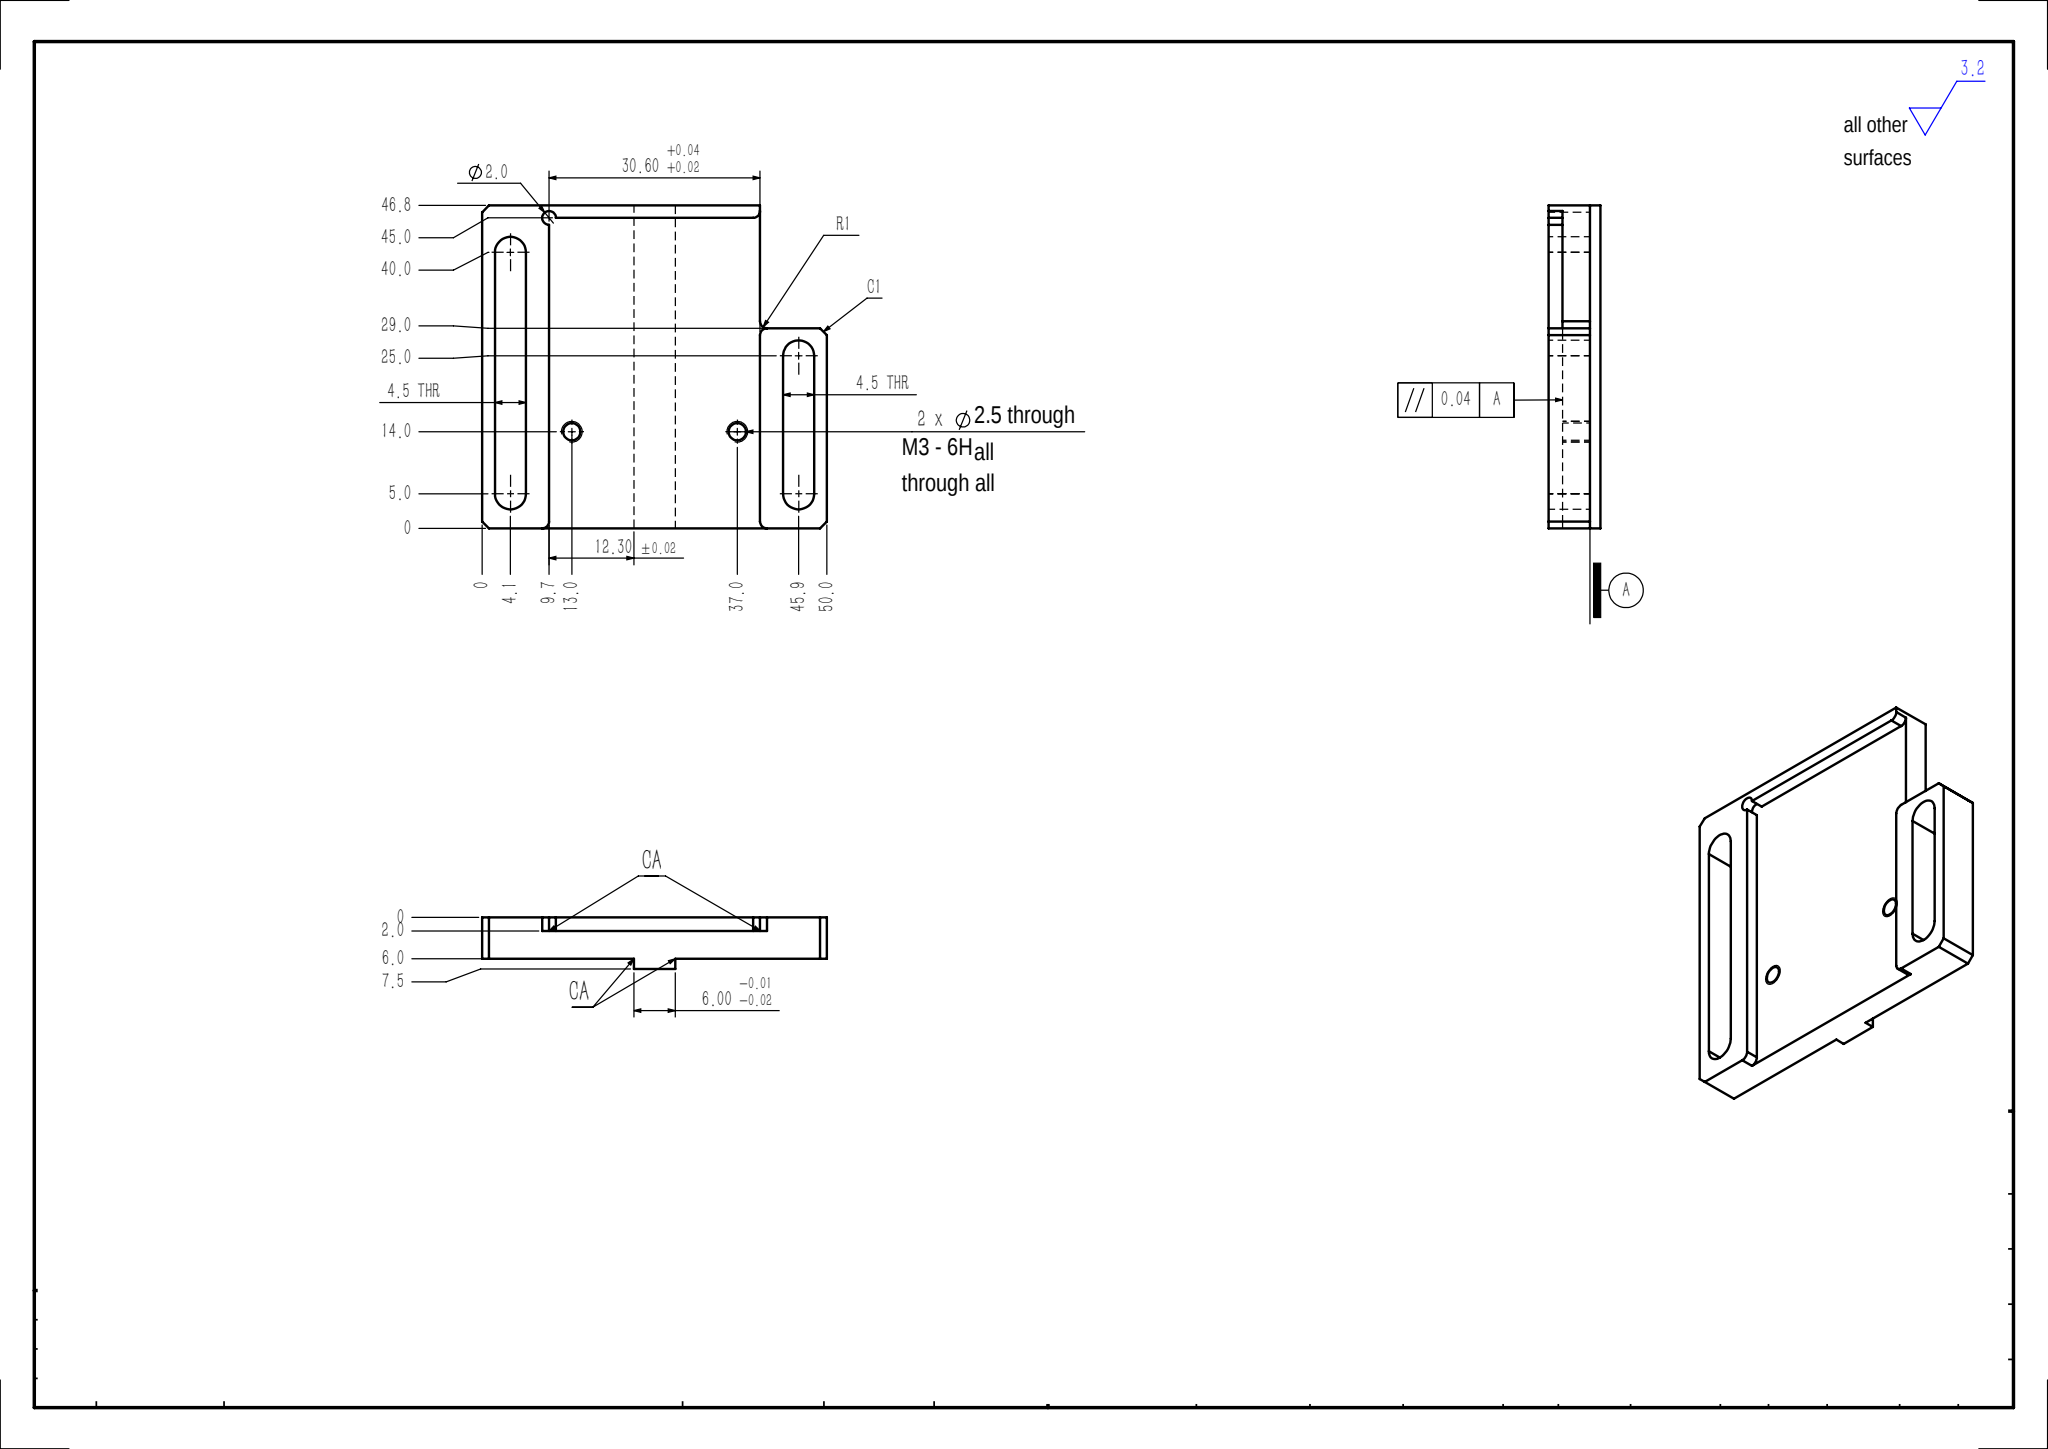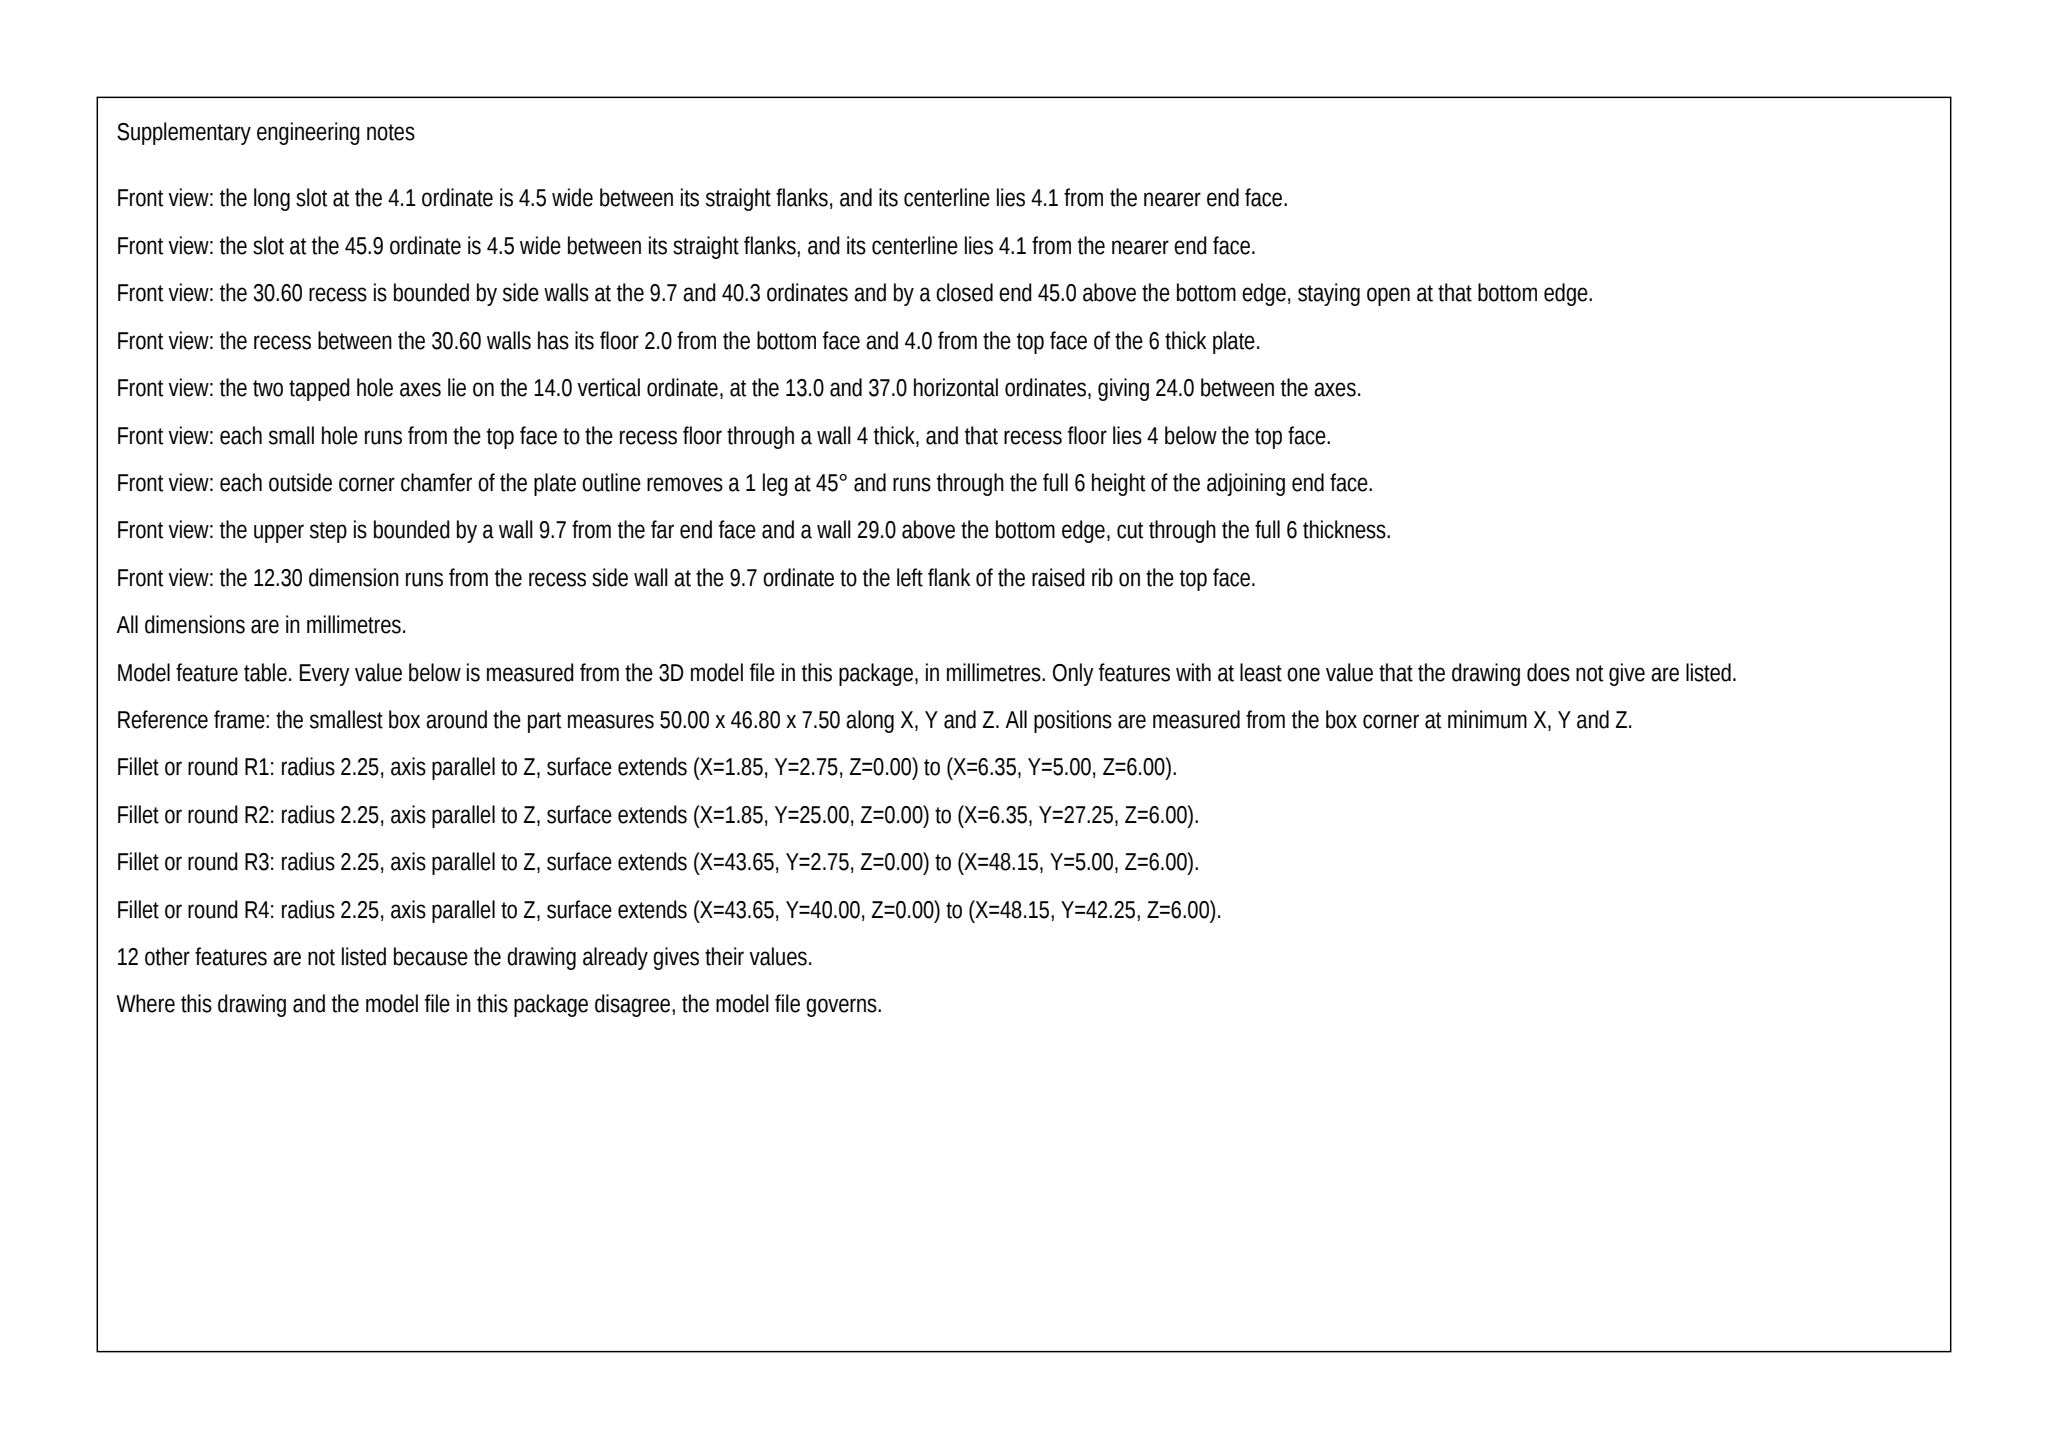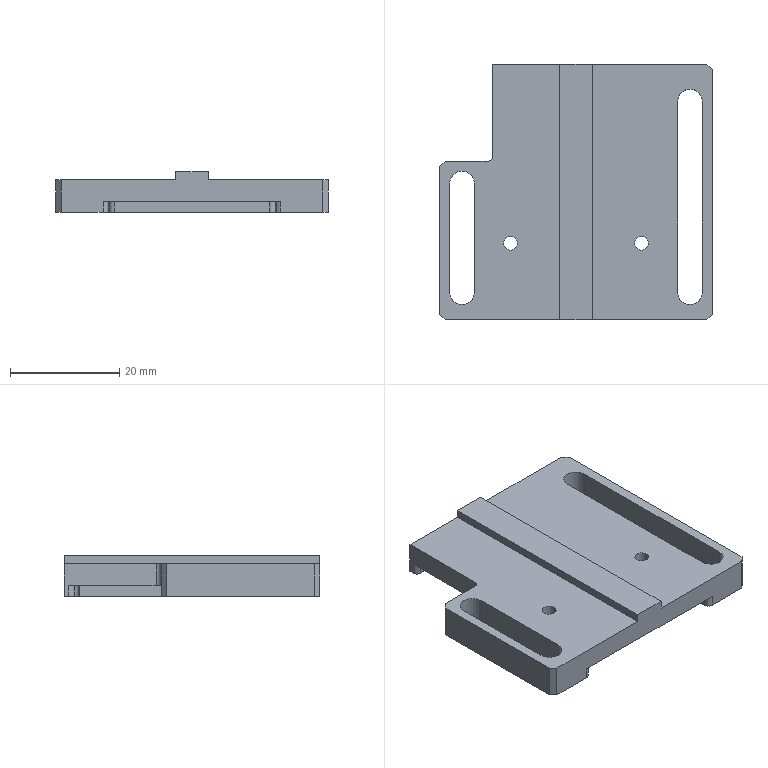Part | SolidWorks | mm | 1 solid | 40 faces | box 50 x 46.8 x 7.5 mm | volume 8939 mm3 | plane 25 | cylinder 15 | commonest cylinder face diameters 2 x7 2.5 x4 4.5 x4
Drawing notes:
6X Ø2.0 CORNER RELIEF CUTS (CA) | from the solid: Six Ø2.0 z-axis cylinders at (8.7,1.0),(8.7,28.0),(8.7,30.0),(10.7,46.0),(40.3,45.0),(41.3,1.0)
Ø2.0 RELIEF CL: Y=1.0, 28.0, 30.0, 45.0, 46.0 FROM Y0 | from the solid: Ø2.0 cylinder pos_other_axes y values 1.0, 28.0, 30.0, 45.0, 46.0 from bbox min y (drawing 0 datum)
Ø2.0 RELIEF X CL: 8.7, 10.7, 40.3, 41.3 FROM X0 | from the solid: Ø2.0 cylinder x positions 8.7, 10.7, 40.3, 41.3 from bbox min x (drawing 0 datum)
Ø2.0 RELIEF DP 2.0 TYP; DP 4.0 AT X8.7 / Y30.0 | from the solid: Ø2.0 cylinder lengths: 2.0 for five, 4.0 for the one at (8.7,30.0)
CA = Ø2.0 CORNER RELIEF, DP 2.0 UNO, SEE FRONT VIEW | from the solid: CA labels in section coincide with Ø2.0 z-axis relief cylinders, length 2.0
RELIEF AXIAL LEN 2.0 AT X9.7 & X40.3 STEP EDGES | from the solid: Ø2.0 cylinders tangent to planes x=9.7 and x=40.3, cylinder length 2.0
build123d program:
from build123d import *

# Parameters (mm, degrees)
SKETCH1_W           = 50
SKETCH1_H           = 47
BOSS_EXTRUDE1_DEPTH = 3
SKETCH2_W           = 30.6
SKETCH2_H           = 45
CUT_EXTRUDE1_DEPTH  = 2
SKETCH3_R           = 1
CUT_EXTRUDE2_DEPTH  = 35.543
SKETCH4_W           = 9.7
SKETCH4_H           = 18
CUT_EXTRUDE3_DEPTH  = 35.832
CUT_EXTRUDE4_DEPTH  = 35.832
SKETCH6_W           = 40.3
SKETCH6_H           = 6
CUT_EXTRUDE5_DEPTH  = 0.2
M3_TAPPED_HOLE1_D   = 2.5
SKETCH9_W           = 6
SKETCH9_H           = 46.8
BOSS_EXTRUDE2_DEPTH = 1.5
FILLET1_R           = 1
FILLET2_R           = 1
CHAMFER1_SIZE       = 1


with BuildPart() as part:
    # Sketch1 → Boss-Extrude1 (new, symmetric)
    with BuildSketch(Plane.XY):
        Rectangle(SKETCH1_W, SKETCH1_H)
    extrude(amount=BOSS_EXTRUDE1_DEPTH, both=True)

    # Sketch2 → Cut-Extrude1 (cut)
    with BuildSketch(Plane(origin=(0, 0, -3), x_dir=(-1, 0, 0), z_dir=(0, 0, -1))):
        with Locations((0, -1)):
            Rectangle(SKETCH2_W, SKETCH2_H)
    extrude(amount=-CUT_EXTRUDE1_DEPTH, mode=Mode.SUBTRACT)

    # Sketch3 → Cut-Extrude2 (cut, through all)
    with BuildSketch(Plane(origin=(0, 0, -1), x_dir=(-1, 0, 0), z_dir=(0, 0, -1))):
        with Locations((-15.3, 21.5)):
            Circle(SKETCH3_R)
    extrude(amount=CUT_EXTRUDE2_DEPTH, mode=Mode.SUBTRACT)

    # Sketch4 → Cut-Extrude3 (cut, through all)
    with BuildSketch(Plane(origin=(0, 0, -3), x_dir=(-1, 0, 0), z_dir=(0, 0, -1))):
        with Locations((20.15, 14.5)):
            Rectangle(SKETCH4_W, SKETCH4_H)
    extrude(amount=-CUT_EXTRUDE3_DEPTH, mode=Mode.SUBTRACT)

    # Sketch5 → Cut-Extrude4 (cut, through all)
    with BuildSketch(Plane(origin=(0, 0, -3), x_dir=(-1, 0, 0), z_dir=(0, 0, -1))):
        with BuildLine():
            Line((18.65, -18.5), (18.65, 1.5))
            ThreePointArc((18.65, 1.5), (20.9, 3.75), (23.15, 1.5))
            Line((23.15, 1.5), (23.15, -18.5))
            ThreePointArc((23.15, -18.5), (20.9, -20.75), (18.65, -18.5))
        make_face()
        with BuildLine():
            Line((-23.15, -18.5), (-23.15, 16.5))
            ThreePointArc((-23.15, 16.5), (-20.9, 18.75), (-18.65, 16.5))
            Line((-18.65, 16.5), (-18.65, -18.5))
            ThreePointArc((-18.65, -18.5), (-20.9, -20.75), (-23.15, -18.5))
        make_face()
    extrude(amount=-CUT_EXTRUDE4_DEPTH, mode=Mode.SUBTRACT)

    # Sketch6 → Cut-Extrude5 (cut)
    with BuildSketch(Plane(origin=(0, 23.5, 0), x_dir=(1, 0, 0), z_dir=(0, 1, 0))):
        with Locations((4.85, 0)):
            Rectangle(SKETCH6_W, SKETCH6_H)
    extrude(amount=-CUT_EXTRUDE5_DEPTH, mode=Mode.SUBTRACT)

    # M3 Tapped Hole1 (through all)
    with Locations(Plane(origin=(0, 0, -1), x_dir=(-1, 0, 0), z_dir=(0, 0, -1))):
        with Locations((12, -9.5), (-12, -9.5)):
            Hole(M3_TAPPED_HOLE1_D / 2)

    # Sketch9 → Boss-Extrude2 (add)
    with BuildSketch(Plane.XY.offset(3)):
        with Locations((0, -0.1)):
            Rectangle(SKETCH9_W, SKETCH9_H)
    extrude(amount=BOSS_EXTRUDE2_DEPTH)

    # Fillet1
    fillet1_edges = [part.edges().sort_by_distance(p)[0] for p in [
        (15.3, -23.5, -2),
        (-15.3, 21.5, -2),
        (-15.3, -23.5, -2),
        (-15.3, 5.5, -2),
    ]]
    fillet(fillet1_edges, radius=FILLET1_R)

    # Fillet2
    fillet2_edges = [part.edges().sort_by_distance(p)[0] for p in [
        (-15.3, 5.5, 1),
    ]]
    fillet(fillet2_edges, radius=FILLET2_R)

    # Chamfer1
    chamfer1_edges = [part.edges().sort_by_distance(p)[0] for p in [
        (-25, 5.5, 0),
        (25, -23.5, 0),
        (-25, -23.5, 0),
        (25, 23.3, 0),
    ]]
    chamfer(chamfer1_edges, length=CHAMFER1_SIZE)


solid = part.part